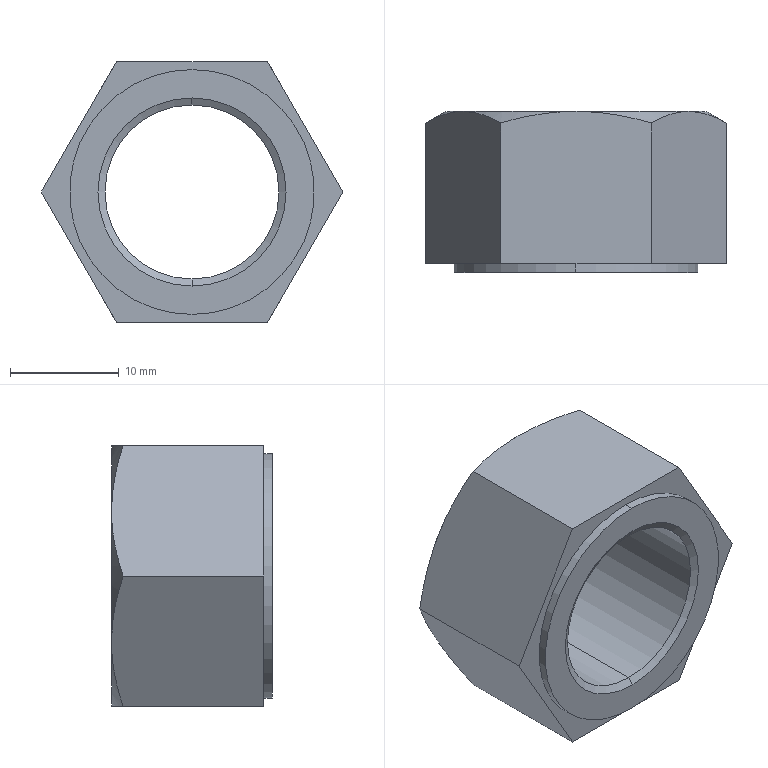Component | SolidWorks | GB_T6170-2015[Type1HexNutM16]-1 | 1 solid | 23 faces | box 27.71 x 14.8 x 24 mm | volume 4298 mm3 | cone 10 | plane 9 | cylinder 4 | commonest cylinder face diameters 22.5 x2 16 x2
STEP:
#1=COLOUR_RGB('',0.7922,0.8196,0.9333);
#2=FILL_AREA_STYLE_COLOUR('',#1);
#3=FILL_AREA_STYLE('',(#2));
#4=SURFACE_STYLE_FILL_AREA(#3);
#5=SURFACE_SIDE_STYLE('',(#4));
#6=SURFACE_STYLE_USAGE(.BOTH.,#5);
#7=PRESENTATION_STYLE_ASSIGNMENT((#6));
#8=CARTESIAN_POINT('',(5.257,-7.433,24.065));
#9=VERTEX_POINT('',#8);
#10=CARTESIAN_POINT('',(5.257,-7.433,23.179));
#11=VERTEX_POINT('',#10);
#12=CARTESIAN_POINT('',(5.257,-7.433,23.622));
#13=DIRECTION('',(-0.,1.,0.));
#14=DIRECTION('',(-0.,-0.,1.));
#15=AXIS2_PLACEMENT_3D('',#12,#13,#14);
#16=CIRCLE('',#15,0.4429);
#17=EDGE_CURVE('',#9,#11,#16,.T.);
#18=ORIENTED_EDGE('',*,*,#17,.T.);
#19=CARTESIAN_POINT('',(5.257,-7.401,23.179));
#20=VERTEX_POINT('',#19);
#21=CARTESIAN_POINT('',(5.257,-6.85,23.179));
#22=DIRECTION('',(-0.,1.,0.));
#23=VECTOR('',#22,39.37);
#24=LINE('',#21,#23);
#25=EDGE_CURVE('',#11,#20,#24,.T.);
#26=ORIENTED_EDGE('',*,*,#25,.T.);
#27=CARTESIAN_POINT('',(5.257,-7.401,24.065));
#28=VERTEX_POINT('',#27);
#29=CARTESIAN_POINT('',(5.257,-7.401,23.622));
#30=DIRECTION('',(-0.,1.,0.));
#31=DIRECTION('',(-0.,-0.,1.));
#32=AXIS2_PLACEMENT_3D('',#29,#30,#31);
#33=CIRCLE('',#32,0.4429);
#34=EDGE_CURVE('',#28,#20,#33,.T.);
#35=ORIENTED_EDGE('',*,*,#34,.F.);
#36=CARTESIAN_POINT('',(5.257,-6.85,24.065));
#37=DIRECTION('',(-0.,1.,0.));
#38=VECTOR('',#37,39.37);
#39=LINE('',#36,#38);
#40=EDGE_CURVE('',#9,#28,#39,.T.);
#41=ORIENTED_EDGE('',*,*,#40,.F.);
#42=EDGE_LOOP('',(#18,#26,#35,#41));
#43=FACE_OUTER_BOUND('',#42,.T.);
#44=CARTESIAN_POINT('',(5.257,-6.85,23.622));
#45=DIRECTION('',(-0.,1.,0.));
#46=DIRECTION('',(-0.,-0.,1.));
#47=AXIS2_PLACEMENT_3D('',#44,#45,#46);
#48=CYLINDRICAL_SURFACE('',#47,0.4429);
#49=ADVANCED_FACE('',(#43),#48,.T.);
#50=CARTESIAN_POINT('',(5.257,-7.418,23.307));
#51=VERTEX_POINT('',#50);
#52=CARTESIAN_POINT('',(5.257,-7.418,23.937));
#53=VERTEX_POINT('',#52);
#54=CARTESIAN_POINT('',(5.257,-7.418,23.622));
#55=DIRECTION('',(-0.,1.,0.));
#56=DIRECTION('',(0.,0.,-1.));
#57=AXIS2_PLACEMENT_3D('',#54,#55,#56);
#58=CIRCLE('',#57,0.315);
#59=EDGE_CURVE('',#51,#53,#58,.T.);
#60=ORIENTED_EDGE('',*,*,#59,.T.);
#61=CARTESIAN_POINT('',(5.257,-7.433,23.963));
#62=VERTEX_POINT('',#61);
#63=CARTESIAN_POINT('',(5.257,-7.433,23.963));
#64=DIRECTION('',(-0.,-0.5,0.866));
#65=VECTOR('',#64,39.37);
#66=LINE('',#63,#65);
#67=EDGE_CURVE('',#53,#62,#66,.T.);
#68=ORIENTED_EDGE('',*,*,#67,.T.);
#69=CARTESIAN_POINT('',(5.257,-7.433,23.281));
#70=VERTEX_POINT('',#69);
#71=CARTESIAN_POINT('',(5.257,-7.433,23.622));
#72=DIRECTION('',(-0.,1.,0.));
#73=DIRECTION('',(-0.,-0.,1.));
#74=AXIS2_PLACEMENT_3D('',#71,#72,#73);
#75=CIRCLE('',#74,0.3406);
#76=EDGE_CURVE('',#70,#62,#75,.T.);
#77=ORIENTED_EDGE('',*,*,#76,.F.);
#78=CARTESIAN_POINT('',(5.257,-7.433,23.281));
#79=DIRECTION('',(0.,-0.5,-0.866));
#80=VECTOR('',#79,39.37);
#81=LINE('',#78,#80);
#82=EDGE_CURVE('',#51,#70,#81,.T.);
#83=ORIENTED_EDGE('',*,*,#82,.F.);
#84=EDGE_LOOP('',(#60,#68,#77,#83));
#85=FACE_OUTER_BOUND('',#84,.T.);
#86=CARTESIAN_POINT('',(5.257,-7.433,23.622));
#87=DIRECTION('',(0.,-1.,-0.));
#88=DIRECTION('',(0.,0.,-1.));
#89=AXIS2_PLACEMENT_3D('',#86,#87,#88);
#90=CONICAL_SURFACE('',#89,0.3406,1.047);
#91=ADVANCED_FACE('',(#85),#90,.F.);
#92=CARTESIAN_POINT('',(5.257,-6.865,23.937));
#93=VERTEX_POINT('',#92);
#94=CARTESIAN_POINT('',(5.257,-6.865,23.307));
#95=VERTEX_POINT('',#94);
#96=CARTESIAN_POINT('',(5.257,-6.865,23.622));
#97=DIRECTION('',(0.,-1.,-0.));
#98=DIRECTION('',(-0.,-0.,1.));
#99=AXIS2_PLACEMENT_3D('',#96,#97,#98);
#100=CIRCLE('',#99,0.315);
#101=EDGE_CURVE('',#93,#95,#100,.T.);
#102=ORIENTED_EDGE('',*,*,#101,.T.);
#103=CARTESIAN_POINT('',(5.257,-6.85,23.281));
#104=VERTEX_POINT('',#103);
#105=CARTESIAN_POINT('',(5.257,-6.889,23.35));
#106=DIRECTION('',(0.,0.5,-0.866));
#107=VECTOR('',#106,39.37);
#108=LINE('',#105,#107);
#109=EDGE_CURVE('',#95,#104,#108,.T.);
#110=ORIENTED_EDGE('',*,*,#109,.T.);
#111=CARTESIAN_POINT('',(5.257,-6.85,23.963));
#112=VERTEX_POINT('',#111);
#113=CARTESIAN_POINT('',(5.257,-6.85,23.622));
#114=DIRECTION('',(-0.,1.,0.));
#115=DIRECTION('',(-0.,-0.,1.));
#116=AXIS2_PLACEMENT_3D('',#113,#114,#115);
#117=CIRCLE('',#116,0.3406);
#118=EDGE_CURVE('',#104,#112,#117,.T.);
#119=ORIENTED_EDGE('',*,*,#118,.T.);
#120=CARTESIAN_POINT('',(5.257,-6.889,23.894));
#121=DIRECTION('',(-0.,0.5,0.866));
#122=VECTOR('',#121,39.37);
#123=LINE('',#120,#122);
#124=EDGE_CURVE('',#93,#112,#123,.T.);
#125=ORIENTED_EDGE('',*,*,#124,.F.);
#126=EDGE_LOOP('',(#102,#110,#119,#125));
#127=FACE_OUTER_BOUND('',#126,.T.);
#128=CARTESIAN_POINT('',(5.257,-6.889,23.622));
#129=DIRECTION('',(-0.,1.,0.));
#130=DIRECTION('',(-0.,-0.,1.));
#131=AXIS2_PLACEMENT_3D('',#128,#129,#130);
#132=CONICAL_SURFACE('',#131,0.2723,1.047);
#133=ADVANCED_FACE('',(#127),#132,.F.);
#134=ORIENTED_EDGE('',*,*,#59,.F.);
#135=CARTESIAN_POINT('',(5.257,-7.433,23.307));
#136=DIRECTION('',(-0.,1.,0.));
#137=VECTOR('',#136,39.37);
#138=LINE('',#135,#137);
#139=EDGE_CURVE('',#51,#95,#138,.T.);
#140=ORIENTED_EDGE('',*,*,#139,.T.);
#141=ORIENTED_EDGE('',*,*,#101,.F.);
#142=CARTESIAN_POINT('',(5.257,-7.433,23.937));
#143=DIRECTION('',(-0.,1.,0.));
#144=VECTOR('',#143,39.37);
#145=LINE('',#142,#144);
#146=EDGE_CURVE('',#53,#93,#145,.T.);
#147=ORIENTED_EDGE('',*,*,#146,.F.);
#148=EDGE_LOOP('',(#134,#140,#141,#147));
#149=FACE_OUTER_BOUND('',#148,.T.);
#150=CARTESIAN_POINT('',(5.257,-7.433,23.622));
#151=DIRECTION('',(-0.,1.,0.));
#152=DIRECTION('',(-0.,-0.,1.));
#153=AXIS2_PLACEMENT_3D('',#150,#151,#152);
#154=CYLINDRICAL_SURFACE('',#153,0.315);
#155=ADVANCED_FACE('',(#149),#154,.F.);
#156=CARTESIAN_POINT('',(5.53,-7.401,24.094));
#157=VERTEX_POINT('',#156);
#158=CARTESIAN_POINT('',(5.53,-6.892,24.094));
#159=VERTEX_POINT('',#158);
#160=CARTESIAN_POINT('',(5.53,-7.433,24.094));
#161=DIRECTION('',(-0.,1.,0.));
#162=VECTOR('',#161,39.37);
#163=LINE('',#160,#162);
#164=EDGE_CURVE('',#157,#159,#163,.T.);
#165=ORIENTED_EDGE('',*,*,#164,.F.);
#166=CARTESIAN_POINT('',(5.803,-7.401,23.622));
#167=VERTEX_POINT('',#166);
#168=CARTESIAN_POINT('',(5.53,-7.401,24.094));
#169=DIRECTION('',(0.5,0.,-0.866));
#170=VECTOR('',#169,39.37);
#171=LINE('',#168,#170);
#172=EDGE_CURVE('',#157,#167,#171,.T.);
#173=ORIENTED_EDGE('',*,*,#172,.T.);
#174=CARTESIAN_POINT('',(5.803,-6.892,23.622));
#175=VERTEX_POINT('',#174);
#176=CARTESIAN_POINT('',(5.803,-7.433,23.622));
#177=DIRECTION('',(-0.,1.,0.));
#178=VECTOR('',#177,39.37);
#179=LINE('',#176,#178);
#180=EDGE_CURVE('',#167,#175,#179,.T.);
#181=ORIENTED_EDGE('',*,*,#180,.T.);
#182=CARTESIAN_POINT('',(5.666,-6.85,23.858));
#183=VERTEX_POINT('',#182);
#184=CARTESIAN_POINT('',(5.803,-6.892,23.622));
#185=CARTESIAN_POINT('',(5.78,-6.879,23.661));
#186=CARTESIAN_POINT('',(5.758,-6.869,23.7));
#187=CARTESIAN_POINT('',(5.712,-6.854,23.778));
#188=CARTESIAN_POINT('',(5.689,-6.85,23.818));
#189=CARTESIAN_POINT('',(5.666,-6.85,23.858));
#190=B_SPLINE_CURVE_WITH_KNOTS('',3,(#184,#185,#186,#187,#188,#189),.UNSPECIFIED.,.F.,.F.,(4,2,4),(0.00000024,0.003505,0.00701),.UNSPECIFIED.);
#191=EDGE_CURVE('',#175,#183,#190,.T.);
#192=ORIENTED_EDGE('',*,*,#191,.T.);
#193=CARTESIAN_POINT('',(5.666,-6.85,23.858));
#194=CARTESIAN_POINT('',(5.655,-6.85,23.878));
#195=CARTESIAN_POINT('',(5.643,-6.851,23.898));
#196=CARTESIAN_POINT('',(5.62,-6.855,23.938));
#197=CARTESIAN_POINT('',(5.609,-6.858,23.958));
#198=CARTESIAN_POINT('',(5.575,-6.869,24.017));
#199=CARTESIAN_POINT('',(5.552,-6.879,24.056));
#200=CARTESIAN_POINT('',(5.53,-6.892,24.094));
#201=B_SPLINE_CURVE_WITH_KNOTS('',3,(#193,#194,#195,#196,#197,#198,#199,#200),.UNSPECIFIED.,.F.,.F.,(4,2,2,4),(0.00701,0.008756,0.0105,0.01399),.UNSPECIFIED.);
#202=EDGE_CURVE('',#183,#159,#201,.T.);
#203=ORIENTED_EDGE('',*,*,#202,.T.);
#204=EDGE_LOOP('',(#165,#173,#181,#192,#203));
#205=FACE_OUTER_BOUND('',#204,.T.);
#206=CARTESIAN_POINT('',(5.53,-7.433,24.094));
#207=DIRECTION('',(0.866,0.,0.5));
#208=DIRECTION('',(0.5,0.,-0.866));
#209=AXIS2_PLACEMENT_3D('',#206,#207,#208);
#210=PLANE('',#209);
#211=ADVANCED_FACE('',(#205),#210,.T.);
#212=CARTESIAN_POINT('',(4.984,-7.401,24.094));
#213=VERTEX_POINT('',#212);
#214=CARTESIAN_POINT('',(4.984,-6.892,24.094));
#215=VERTEX_POINT('',#214);
#216=CARTESIAN_POINT('',(4.984,-7.433,24.094));
#217=DIRECTION('',(-0.,1.,0.));
#218=VECTOR('',#217,39.37);
#219=LINE('',#216,#218);
#220=EDGE_CURVE('',#213,#215,#219,.T.);
#221=ORIENTED_EDGE('',*,*,#220,.F.);
#222=CARTESIAN_POINT('',(4.984,-7.401,24.094));
#223=DIRECTION('',(1.,0.,0.));
#224=VECTOR('',#223,39.37);
#225=LINE('',#222,#224);
#226=EDGE_CURVE('',#213,#157,#225,.T.);
#227=ORIENTED_EDGE('',*,*,#226,.T.);
#228=ORIENTED_EDGE('',*,*,#164,.T.);
#229=CARTESIAN_POINT('',(5.257,-6.85,24.094));
#230=VERTEX_POINT('',#229);
#231=CARTESIAN_POINT('',(5.53,-6.892,24.094));
#232=CARTESIAN_POINT('',(5.486,-6.879,24.094));
#233=CARTESIAN_POINT('',(5.441,-6.869,24.094));
#234=CARTESIAN_POINT('',(5.373,-6.858,24.094));
#235=CARTESIAN_POINT('',(5.35,-6.855,24.094));
#236=CARTESIAN_POINT('',(5.303,-6.851,24.094));
#237=CARTESIAN_POINT('',(5.28,-6.85,24.094));
#238=CARTESIAN_POINT('',(5.257,-6.85,24.094));
#239=B_SPLINE_CURVE_WITH_KNOTS('',3,(#231,#232,#233,#234,#235,#236,#237,#238),.UNSPECIFIED.,.F.,.F.,(4,2,2,4),(0.03088,0.03439,0.03615,0.0379),.UNSPECIFIED.);
#240=EDGE_CURVE('',#159,#230,#239,.T.);
#241=ORIENTED_EDGE('',*,*,#240,.T.);
#242=CARTESIAN_POINT('',(5.257,-6.85,24.094));
#243=CARTESIAN_POINT('',(5.211,-6.85,24.094));
#244=CARTESIAN_POINT('',(5.165,-6.854,24.094));
#245=CARTESIAN_POINT('',(5.074,-6.869,24.094));
#246=CARTESIAN_POINT('',(5.029,-6.879,24.094));
#247=CARTESIAN_POINT('',(4.984,-6.892,24.094));
#248=B_SPLINE_CURVE_WITH_KNOTS('',3,(#242,#243,#244,#245,#246,#247),.UNSPECIFIED.,.F.,.F.,(4,2,4),(0.0379,0.04141,0.04492),.UNSPECIFIED.);
#249=EDGE_CURVE('',#230,#215,#248,.T.);
#250=ORIENTED_EDGE('',*,*,#249,.T.);
#251=EDGE_LOOP('',(#221,#227,#228,#241,#250));
#252=FACE_OUTER_BOUND('',#251,.T.);
#253=CARTESIAN_POINT('',(4.984,-7.433,24.094));
#254=DIRECTION('',(-0.,-0.,1.));
#255=DIRECTION('',(0.,-1.,-0.));
#256=AXIS2_PLACEMENT_3D('',#253,#254,#255);
#257=PLANE('',#256);
#258=ADVANCED_FACE('',(#252),#257,.T.);
#259=CARTESIAN_POINT('',(4.712,-7.401,23.622));
#260=VERTEX_POINT('',#259);
#261=CARTESIAN_POINT('',(4.712,-6.892,23.622));
#262=VERTEX_POINT('',#261);
#263=CARTESIAN_POINT('',(4.712,-7.433,23.622));
#264=DIRECTION('',(-0.,1.,0.));
#265=VECTOR('',#264,39.37);
#266=LINE('',#263,#265);
#267=EDGE_CURVE('',#260,#262,#266,.T.);
#268=ORIENTED_EDGE('',*,*,#267,.F.);
#269=CARTESIAN_POINT('',(4.712,-7.401,23.622));
#270=DIRECTION('',(0.5,0.,0.866));
#271=VECTOR('',#270,39.37);
#272=LINE('',#269,#271);
#273=EDGE_CURVE('',#260,#213,#272,.T.);
#274=ORIENTED_EDGE('',*,*,#273,.T.);
#275=ORIENTED_EDGE('',*,*,#220,.T.);
#276=CARTESIAN_POINT('',(4.848,-6.85,23.858));
#277=VERTEX_POINT('',#276);
#278=CARTESIAN_POINT('',(4.984,-6.892,24.094));
#279=CARTESIAN_POINT('',(4.962,-6.879,24.056));
#280=CARTESIAN_POINT('',(4.94,-6.869,24.017));
#281=CARTESIAN_POINT('',(4.894,-6.854,23.938));
#282=CARTESIAN_POINT('',(4.871,-6.85,23.899));
#283=CARTESIAN_POINT('',(4.848,-6.85,23.858));
#284=B_SPLINE_CURVE_WITH_KNOTS('',3,(#278,#279,#280,#281,#282,#283),.UNSPECIFIED.,.F.,.F.,(4,2,4),(0.00000024,0.003505,0.00701),.UNSPECIFIED.);
#285=EDGE_CURVE('',#215,#277,#284,.T.);
#286=ORIENTED_EDGE('',*,*,#285,.T.);
#287=CARTESIAN_POINT('',(4.848,-6.85,23.858));
#288=CARTESIAN_POINT('',(4.836,-6.85,23.838));
#289=CARTESIAN_POINT('',(4.825,-6.851,23.818));
#290=CARTESIAN_POINT('',(4.802,-6.855,23.778));
#291=CARTESIAN_POINT('',(4.79,-6.858,23.758));
#292=CARTESIAN_POINT('',(4.756,-6.869,23.699));
#293=CARTESIAN_POINT('',(4.734,-6.879,23.661));
#294=CARTESIAN_POINT('',(4.712,-6.892,23.622));
#295=B_SPLINE_CURVE_WITH_KNOTS('',3,(#287,#288,#289,#290,#291,#292,#293,#294),.UNSPECIFIED.,.F.,.F.,(4,2,2,4),(0.00701,0.008756,0.0105,0.01399),.UNSPECIFIED.);
#296=EDGE_CURVE('',#277,#262,#295,.T.);
#297=ORIENTED_EDGE('',*,*,#296,.T.);
#298=EDGE_LOOP('',(#268,#274,#275,#286,#297));
#299=FACE_OUTER_BOUND('',#298,.T.);
#300=CARTESIAN_POINT('',(4.712,-7.433,23.622));
#301=DIRECTION('',(-0.866,-0.,0.5));
#302=DIRECTION('',(0.5,0.,0.866));
#303=AXIS2_PLACEMENT_3D('',#300,#301,#302);
#304=PLANE('',#303);
#305=ADVANCED_FACE('',(#299),#304,.T.);
#306=CARTESIAN_POINT('',(4.984,-7.401,23.15));
#307=VERTEX_POINT('',#306);
#308=CARTESIAN_POINT('',(4.984,-6.892,23.15));
#309=VERTEX_POINT('',#308);
#310=CARTESIAN_POINT('',(4.984,-7.433,23.15));
#311=DIRECTION('',(-0.,1.,0.));
#312=VECTOR('',#311,39.37);
#313=LINE('',#310,#312);
#314=EDGE_CURVE('',#307,#309,#313,.T.);
#315=ORIENTED_EDGE('',*,*,#314,.F.);
#316=CARTESIAN_POINT('',(4.984,-7.401,23.15));
#317=DIRECTION('',(-0.5,-0.,0.866));
#318=VECTOR('',#317,39.37);
#319=LINE('',#316,#318);
#320=EDGE_CURVE('',#307,#260,#319,.T.);
#321=ORIENTED_EDGE('',*,*,#320,.T.);
#322=ORIENTED_EDGE('',*,*,#267,.T.);
#323=CARTESIAN_POINT('',(4.848,-6.85,23.386));
#324=VERTEX_POINT('',#323);
#325=CARTESIAN_POINT('',(4.712,-6.892,23.622));
#326=CARTESIAN_POINT('',(4.734,-6.879,23.583));
#327=CARTESIAN_POINT('',(4.756,-6.869,23.544));
#328=CARTESIAN_POINT('',(4.802,-6.854,23.466));
#329=CARTESIAN_POINT('',(4.825,-6.85,23.426));
#330=CARTESIAN_POINT('',(4.848,-6.85,23.386));
#331=B_SPLINE_CURVE_WITH_KNOTS('',3,(#325,#326,#327,#328,#329,#330),.UNSPECIFIED.,.F.,.F.,(4,2,4),(0.00000024,0.003505,0.00701),.UNSPECIFIED.);
#332=EDGE_CURVE('',#262,#324,#331,.T.);
#333=ORIENTED_EDGE('',*,*,#332,.T.);
#334=CARTESIAN_POINT('',(4.848,-6.85,23.386));
#335=CARTESIAN_POINT('',(4.859,-6.85,23.366));
#336=CARTESIAN_POINT('',(4.871,-6.851,23.346));
#337=CARTESIAN_POINT('',(4.894,-6.855,23.306));
#338=CARTESIAN_POINT('',(4.906,-6.858,23.286));
#339=CARTESIAN_POINT('',(4.94,-6.869,23.227));
#340=CARTESIAN_POINT('',(4.962,-6.879,23.188));
#341=CARTESIAN_POINT('',(4.984,-6.892,23.15));
#342=B_SPLINE_CURVE_WITH_KNOTS('',3,(#334,#335,#336,#337,#338,#339,#340,#341),.UNSPECIFIED.,.F.,.F.,(4,2,2,4),(0.00701,0.008756,0.0105,0.01399),.UNSPECIFIED.);
#343=EDGE_CURVE('',#324,#309,#342,.T.);
#344=ORIENTED_EDGE('',*,*,#343,.T.);
#345=EDGE_LOOP('',(#315,#321,#322,#333,#344));
#346=FACE_OUTER_BOUND('',#345,.T.);
#347=CARTESIAN_POINT('',(4.984,-7.433,23.15));
#348=DIRECTION('',(-0.866,-0.,-0.5));
#349=DIRECTION('',(-0.5,-0.,0.866));
#350=AXIS2_PLACEMENT_3D('',#347,#348,#349);
#351=PLANE('',#350);
#352=ADVANCED_FACE('',(#346),#351,.T.);
#353=CARTESIAN_POINT('',(5.53,-7.401,23.15));
#354=VERTEX_POINT('',#353);
#355=CARTESIAN_POINT('',(5.53,-6.892,23.15));
#356=VERTEX_POINT('',#355);
#357=CARTESIAN_POINT('',(5.53,-7.433,23.15));
#358=DIRECTION('',(-0.,1.,0.));
#359=VECTOR('',#358,39.37);
#360=LINE('',#357,#359);
#361=EDGE_CURVE('',#354,#356,#360,.T.);
#362=ORIENTED_EDGE('',*,*,#361,.F.);
#363=CARTESIAN_POINT('',(5.53,-7.401,23.15));
#364=DIRECTION('',(-1.,-0.,-0.));
#365=VECTOR('',#364,39.37);
#366=LINE('',#363,#365);
#367=EDGE_CURVE('',#354,#307,#366,.T.);
#368=ORIENTED_EDGE('',*,*,#367,.T.);
#369=ORIENTED_EDGE('',*,*,#314,.T.);
#370=CARTESIAN_POINT('',(5.257,-6.85,23.15));
#371=VERTEX_POINT('',#370);
#372=CARTESIAN_POINT('',(4.984,-6.892,23.15));
#373=CARTESIAN_POINT('',(5.029,-6.879,23.15));
#374=CARTESIAN_POINT('',(5.074,-6.869,23.15));
#375=CARTESIAN_POINT('',(5.165,-6.854,23.15));
#376=CARTESIAN_POINT('',(5.211,-6.85,23.15));
#377=CARTESIAN_POINT('',(5.257,-6.85,23.15));
#378=B_SPLINE_CURVE_WITH_KNOTS('',3,(#372,#373,#374,#375,#376,#377),.UNSPECIFIED.,.F.,.F.,(4,2,4),(0.01255,0.01606,0.01957),.UNSPECIFIED.);
#379=EDGE_CURVE('',#309,#371,#378,.T.);
#380=ORIENTED_EDGE('',*,*,#379,.T.);
#381=CARTESIAN_POINT('',(5.257,-6.85,23.15));
#382=CARTESIAN_POINT('',(5.28,-6.85,23.15));
#383=CARTESIAN_POINT('',(5.303,-6.851,23.15));
#384=CARTESIAN_POINT('',(5.35,-6.855,23.15));
#385=CARTESIAN_POINT('',(5.373,-6.858,23.15));
#386=CARTESIAN_POINT('',(5.441,-6.869,23.15));
#387=CARTESIAN_POINT('',(5.486,-6.879,23.15));
#388=CARTESIAN_POINT('',(5.53,-6.892,23.15));
#389=B_SPLINE_CURVE_WITH_KNOTS('',3,(#381,#382,#383,#384,#385,#386,#387,#388),.UNSPECIFIED.,.F.,.F.,(4,2,2,4),(0.01957,0.02132,0.02307,0.02658),.UNSPECIFIED.);
#390=EDGE_CURVE('',#371,#356,#389,.T.);
#391=ORIENTED_EDGE('',*,*,#390,.T.);
#392=EDGE_LOOP('',(#362,#368,#369,#380,#391));
#393=FACE_OUTER_BOUND('',#392,.T.);
#394=CARTESIAN_POINT('',(5.53,-7.433,23.15));
#395=DIRECTION('',(0.,0.,-1.));
#396=DIRECTION('',(-0.,1.,0.));
#397=AXIS2_PLACEMENT_3D('',#394,#395,#396);
#398=PLANE('',#397);
#399=ADVANCED_FACE('',(#393),#398,.T.);
#400=ORIENTED_EDGE('',*,*,#180,.F.);
#401=CARTESIAN_POINT('',(5.803,-7.401,23.622));
#402=DIRECTION('',(-0.5,-0.,-0.866));
#403=VECTOR('',#402,39.37);
#404=LINE('',#401,#403);
#405=EDGE_CURVE('',#167,#354,#404,.T.);
#406=ORIENTED_EDGE('',*,*,#405,.T.);
#407=ORIENTED_EDGE('',*,*,#361,.T.);
#408=CARTESIAN_POINT('',(5.666,-6.85,23.386));
#409=VERTEX_POINT('',#408);
#410=CARTESIAN_POINT('',(5.53,-6.892,23.15));
#411=CARTESIAN_POINT('',(5.552,-6.879,23.188));
#412=CARTESIAN_POINT('',(5.575,-6.869,23.227));
#413=CARTESIAN_POINT('',(5.62,-6.854,23.306));
#414=CARTESIAN_POINT('',(5.643,-6.85,23.346));
#415=CARTESIAN_POINT('',(5.666,-6.85,23.386));
#416=B_SPLINE_CURVE_WITH_KNOTS('',3,(#410,#411,#412,#413,#414,#415),.UNSPECIFIED.,.F.,.F.,(4,2,4),(0.00000024,0.003505,0.00701),.UNSPECIFIED.);
#417=EDGE_CURVE('',#356,#409,#416,.T.);
#418=ORIENTED_EDGE('',*,*,#417,.T.);
#419=CARTESIAN_POINT('',(5.666,-6.85,23.386));
#420=CARTESIAN_POINT('',(5.678,-6.85,23.406));
#421=CARTESIAN_POINT('',(5.689,-6.851,23.426));
#422=CARTESIAN_POINT('',(5.712,-6.855,23.466));
#423=CARTESIAN_POINT('',(5.724,-6.858,23.486));
#424=CARTESIAN_POINT('',(5.758,-6.869,23.545));
#425=CARTESIAN_POINT('',(5.78,-6.879,23.584));
#426=CARTESIAN_POINT('',(5.803,-6.892,23.622));
#427=B_SPLINE_CURVE_WITH_KNOTS('',3,(#419,#420,#421,#422,#423,#424,#425,#426),.UNSPECIFIED.,.F.,.F.,(4,2,2,4),(0.00701,0.008756,0.0105,0.01399),.UNSPECIFIED.);
#428=EDGE_CURVE('',#409,#175,#427,.T.);
#429=ORIENTED_EDGE('',*,*,#428,.T.);
#430=EDGE_LOOP('',(#400,#406,#407,#418,#429));
#431=FACE_OUTER_BOUND('',#430,.T.);
#432=CARTESIAN_POINT('',(5.803,-7.433,23.622));
#433=DIRECTION('',(0.866,0.,-0.5));
#434=DIRECTION('',(-0.5,-0.,-0.866));
#435=AXIS2_PLACEMENT_3D('',#432,#433,#434);
#436=PLANE('',#435);
#437=ADVANCED_FACE('',(#431),#436,.T.);
#438=ORIENTED_EDGE('',*,*,#76,.T.);
#439=CARTESIAN_POINT('',(5.257,-7.433,23.622));
#440=DIRECTION('',(-0.,1.,0.));
#441=DIRECTION('',(-0.,-0.,1.));
#442=AXIS2_PLACEMENT_3D('',#439,#440,#441);
#443=CIRCLE('',#442,0.3406);
#444=EDGE_CURVE('',#62,#70,#443,.T.);
#445=ORIENTED_EDGE('',*,*,#444,.T.);
#446=EDGE_LOOP('',(#438,#445));
#447=FACE_BOUND('',#446,.T.);
#448=ORIENTED_EDGE('',*,*,#17,.F.);
#449=CARTESIAN_POINT('',(5.257,-7.433,23.622));
#450=DIRECTION('',(-0.,1.,0.));
#451=DIRECTION('',(-0.,-0.,1.));
#452=AXIS2_PLACEMENT_3D('',#449,#450,#451);
#453=CIRCLE('',#452,0.4429);
#454=EDGE_CURVE('',#11,#9,#453,.T.);
#455=ORIENTED_EDGE('',*,*,#454,.F.);
#456=EDGE_LOOP('',(#448,#455));
#457=FACE_OUTER_BOUND('',#456,.T.);
#458=CARTESIAN_POINT('',(5.803,-7.433,23.622));
#459=DIRECTION('',(-0.,1.,0.));
#460=DIRECTION('',(-0.,-0.,1.));
#461=AXIS2_PLACEMENT_3D('',#458,#459,#460);
#462=PLANE('',#461);
#463=ADVANCED_FACE('',(#447,#457),#462,.F.);
#464=CARTESIAN_POINT('',(5.257,-6.85,23.622));
#465=DIRECTION('',(-0.,1.,0.));
#466=DIRECTION('',(-0.,-0.,1.));
#467=AXIS2_PLACEMENT_3D('',#464,#465,#466);
#468=CIRCLE('',#467,0.3406);
#469=EDGE_CURVE('',#112,#104,#468,.T.);
#470=ORIENTED_EDGE('',*,*,#469,.F.);
#471=ORIENTED_EDGE('',*,*,#118,.F.);
#472=EDGE_LOOP('',(#470,#471));
#473=FACE_BOUND('',#472,.T.);
#474=CARTESIAN_POINT('',(5.257,-6.85,23.622));
#475=DIRECTION('',(-0.,1.,0.));
#476=DIRECTION('',(-0.,-0.,1.));
#477=AXIS2_PLACEMENT_3D('',#474,#475,#476);
#478=CIRCLE('',#477,0.4724);
#479=EDGE_CURVE('',#277,#230,#478,.T.);
#480=ORIENTED_EDGE('',*,*,#479,.T.);
#481=CARTESIAN_POINT('',(5.257,-6.85,23.622));
#482=DIRECTION('',(-0.,1.,0.));
#483=DIRECTION('',(-0.,-0.,1.));
#484=AXIS2_PLACEMENT_3D('',#481,#482,#483);
#485=CIRCLE('',#484,0.4724);
#486=EDGE_CURVE('',#230,#183,#485,.T.);
#487=ORIENTED_EDGE('',*,*,#486,.T.);
#488=CARTESIAN_POINT('',(5.257,-6.85,23.622));
#489=DIRECTION('',(-0.,1.,0.));
#490=DIRECTION('',(-0.,-0.,1.));
#491=AXIS2_PLACEMENT_3D('',#488,#489,#490);
#492=CIRCLE('',#491,0.4724);
#493=EDGE_CURVE('',#183,#409,#492,.T.);
#494=ORIENTED_EDGE('',*,*,#493,.T.);
#495=CARTESIAN_POINT('',(5.257,-6.85,23.622));
#496=DIRECTION('',(-0.,1.,0.));
#497=DIRECTION('',(-0.,-0.,1.));
#498=AXIS2_PLACEMENT_3D('',#495,#496,#497);
#499=CIRCLE('',#498,0.4724);
#500=EDGE_CURVE('',#409,#371,#499,.T.);
#501=ORIENTED_EDGE('',*,*,#500,.T.);
#502=CARTESIAN_POINT('',(5.257,-6.85,23.622));
#503=DIRECTION('',(-0.,1.,0.));
#504=DIRECTION('',(-0.,-0.,1.));
#505=AXIS2_PLACEMENT_3D('',#502,#503,#504);
#506=CIRCLE('',#505,0.4724);
#507=EDGE_CURVE('',#371,#324,#506,.T.);
#508=ORIENTED_EDGE('',*,*,#507,.T.);
#509=CARTESIAN_POINT('',(5.257,-6.85,23.622));
#510=DIRECTION('',(-0.,1.,0.));
#511=DIRECTION('',(-0.,-0.,1.));
#512=AXIS2_PLACEMENT_3D('',#509,#510,#511);
#513=CIRCLE('',#512,0.4724);
#514=EDGE_CURVE('',#324,#277,#513,.T.);
#515=ORIENTED_EDGE('',*,*,#514,.T.);
#516=EDGE_LOOP('',(#480,#487,#494,#501,#508,#515));
#517=FACE_OUTER_BOUND('',#516,.T.);
#518=CARTESIAN_POINT('',(5.803,-6.85,23.622));
#519=DIRECTION('',(-0.,1.,0.));
#520=DIRECTION('',(-0.,-0.,1.));
#521=AXIS2_PLACEMENT_3D('',#518,#519,#520);
#522=PLANE('',#521);
#523=ADVANCED_FACE('',(#473,#517),#522,.T.);
#524=ORIENTED_EDGE('',*,*,#139,.F.);
#525=CARTESIAN_POINT('',(5.257,-7.418,23.622));
#526=DIRECTION('',(-0.,1.,0.));
#527=DIRECTION('',(0.,0.,-1.));
#528=AXIS2_PLACEMENT_3D('',#525,#526,#527);
#529=CIRCLE('',#528,0.315);
#530=EDGE_CURVE('',#53,#51,#529,.T.);
#531=ORIENTED_EDGE('',*,*,#530,.F.);
#532=ORIENTED_EDGE('',*,*,#146,.T.);
#533=CARTESIAN_POINT('',(5.257,-6.865,23.622));
#534=DIRECTION('',(0.,-1.,-0.));
#535=DIRECTION('',(-0.,-0.,1.));
#536=AXIS2_PLACEMENT_3D('',#533,#534,#535);
#537=CIRCLE('',#536,0.315);
#538=EDGE_CURVE('',#95,#93,#537,.T.);
#539=ORIENTED_EDGE('',*,*,#538,.F.);
#540=EDGE_LOOP('',(#524,#531,#532,#539));
#541=FACE_OUTER_BOUND('',#540,.T.);
#542=CARTESIAN_POINT('',(5.257,-7.433,23.622));
#543=DIRECTION('',(-0.,1.,0.));
#544=DIRECTION('',(-0.,-0.,1.));
#545=AXIS2_PLACEMENT_3D('',#542,#543,#544);
#546=CYLINDRICAL_SURFACE('',#545,0.315);
#547=ADVANCED_FACE('',(#541),#546,.F.);
#548=ORIENTED_EDGE('',*,*,#109,.F.);
#549=ORIENTED_EDGE('',*,*,#538,.T.);
#550=ORIENTED_EDGE('',*,*,#124,.T.);
#551=ORIENTED_EDGE('',*,*,#469,.T.);
#552=EDGE_LOOP('',(#548,#549,#550,#551));
#553=FACE_OUTER_BOUND('',#552,.T.);
#554=CARTESIAN_POINT('',(5.257,-6.889,23.622));
#555=DIRECTION('',(-0.,1.,0.));
#556=DIRECTION('',(-0.,-0.,1.));
#557=AXIS2_PLACEMENT_3D('',#554,#555,#556);
#558=CONICAL_SURFACE('',#557,0.2723,1.047);
#559=ADVANCED_FACE('',(#553),#558,.F.);
#560=ORIENTED_EDGE('',*,*,#67,.F.);
#561=ORIENTED_EDGE('',*,*,#530,.T.);
#562=ORIENTED_EDGE('',*,*,#82,.T.);
#563=ORIENTED_EDGE('',*,*,#444,.F.);
#564=EDGE_LOOP('',(#560,#561,#562,#563));
#565=FACE_OUTER_BOUND('',#564,.T.);
#566=CARTESIAN_POINT('',(5.257,-7.433,23.622));
#567=DIRECTION('',(0.,-1.,-0.));
#568=DIRECTION('',(0.,0.,-1.));
#569=AXIS2_PLACEMENT_3D('',#566,#567,#568);
#570=CONICAL_SURFACE('',#569,0.3406,1.047);
#571=ADVANCED_FACE('',(#565),#570,.F.);
#572=ORIENTED_EDGE('',*,*,#428,.F.);
#573=ORIENTED_EDGE('',*,*,#493,.F.);
#574=ORIENTED_EDGE('',*,*,#191,.F.);
#575=EDGE_LOOP('',(#572,#573,#574));
#576=FACE_OUTER_BOUND('',#575,.T.);
#577=CARTESIAN_POINT('',(5.257,-6.85,23.622));
#578=DIRECTION('',(0.,-1.,-0.));
#579=DIRECTION('',(-0.,-0.,1.));
#580=AXIS2_PLACEMENT_3D('',#577,#578,#579);
#581=CONICAL_SURFACE('',#580,0.4724,1.047);
#582=ADVANCED_FACE('',(#576),#581,.T.);
#583=ORIENTED_EDGE('',*,*,#500,.F.);
#584=ORIENTED_EDGE('',*,*,#417,.F.);
#585=ORIENTED_EDGE('',*,*,#390,.F.);
#586=EDGE_LOOP('',(#583,#584,#585));
#587=FACE_OUTER_BOUND('',#586,.T.);
#588=CARTESIAN_POINT('',(5.257,-6.85,23.622));
#589=DIRECTION('',(0.,-1.,-0.));
#590=DIRECTION('',(-0.,-0.,1.));
#591=AXIS2_PLACEMENT_3D('',#588,#589,#590);
#592=CONICAL_SURFACE('',#591,0.4724,1.047);
#593=ADVANCED_FACE('',(#587),#592,.T.);
#594=ORIENTED_EDGE('',*,*,#507,.F.);
#595=ORIENTED_EDGE('',*,*,#379,.F.);
#596=ORIENTED_EDGE('',*,*,#343,.F.);
#597=EDGE_LOOP('',(#594,#595,#596));
#598=FACE_OUTER_BOUND('',#597,.T.);
#599=CARTESIAN_POINT('',(5.257,-6.85,23.622));
#600=DIRECTION('',(0.,-1.,-0.));
#601=DIRECTION('',(-0.,-0.,1.));
#602=AXIS2_PLACEMENT_3D('',#599,#600,#601);
#603=CONICAL_SURFACE('',#602,0.4724,1.047);
#604=ADVANCED_FACE('',(#598),#603,.T.);
#605=ORIENTED_EDGE('',*,*,#514,.F.);
#606=ORIENTED_EDGE('',*,*,#332,.F.);
#607=ORIENTED_EDGE('',*,*,#296,.F.);
#608=EDGE_LOOP('',(#605,#606,#607));
#609=FACE_OUTER_BOUND('',#608,.T.);
#610=CARTESIAN_POINT('',(5.257,-6.85,23.622));
#611=DIRECTION('',(0.,-1.,-0.));
#612=DIRECTION('',(-0.,-0.,1.));
#613=AXIS2_PLACEMENT_3D('',#610,#611,#612);
#614=CONICAL_SURFACE('',#613,0.4724,1.047);
#615=ADVANCED_FACE('',(#609),#614,.T.);
#616=ORIENTED_EDGE('',*,*,#479,.F.);
#617=ORIENTED_EDGE('',*,*,#285,.F.);
#618=ORIENTED_EDGE('',*,*,#249,.F.);
#619=EDGE_LOOP('',(#616,#617,#618));
#620=FACE_OUTER_BOUND('',#619,.T.);
#621=CARTESIAN_POINT('',(5.257,-6.85,23.622));
#622=DIRECTION('',(0.,-1.,-0.));
#623=DIRECTION('',(-0.,-0.,1.));
#624=AXIS2_PLACEMENT_3D('',#621,#622,#623);
#625=CONICAL_SURFACE('',#624,0.4724,1.047);
#626=ADVANCED_FACE('',(#620),#625,.T.);
#627=ORIENTED_EDGE('',*,*,#486,.F.);
#628=ORIENTED_EDGE('',*,*,#240,.F.);
#629=ORIENTED_EDGE('',*,*,#202,.F.);
#630=EDGE_LOOP('',(#627,#628,#629));
#631=FACE_OUTER_BOUND('',#630,.T.);
#632=CARTESIAN_POINT('',(5.257,-6.85,23.622));
#633=DIRECTION('',(0.,-1.,-0.));
#634=DIRECTION('',(-0.,-0.,1.));
#635=AXIS2_PLACEMENT_3D('',#632,#633,#634);
#636=CONICAL_SURFACE('',#635,0.4724,1.047);
#637=ADVANCED_FACE('',(#631),#636,.T.);
#638=ORIENTED_EDGE('',*,*,#25,.F.);
#639=ORIENTED_EDGE('',*,*,#454,.T.);
#640=ORIENTED_EDGE('',*,*,#40,.T.);
#641=CARTESIAN_POINT('',(5.257,-7.401,23.622));
#642=DIRECTION('',(-0.,1.,0.));
#643=DIRECTION('',(-0.,-0.,1.));
#644=AXIS2_PLACEMENT_3D('',#641,#642,#643);
#645=CIRCLE('',#644,0.4429);
#646=EDGE_CURVE('',#20,#28,#645,.T.);
#647=ORIENTED_EDGE('',*,*,#646,.F.);
#648=EDGE_LOOP('',(#638,#639,#640,#647));
#649=FACE_OUTER_BOUND('',#648,.T.);
#650=CARTESIAN_POINT('',(5.257,-6.85,23.622));
#651=DIRECTION('',(-0.,1.,0.));
#652=DIRECTION('',(-0.,-0.,1.));
#653=AXIS2_PLACEMENT_3D('',#650,#651,#652);
#654=CYLINDRICAL_SURFACE('',#653,0.4429);
#655=ADVANCED_FACE('',(#649),#654,.T.);
#656=ORIENTED_EDGE('',*,*,#34,.T.);
#657=ORIENTED_EDGE('',*,*,#646,.T.);
#658=EDGE_LOOP('',(#656,#657));
#659=FACE_BOUND('',#658,.T.);
#660=ORIENTED_EDGE('',*,*,#226,.F.);
#661=ORIENTED_EDGE('',*,*,#273,.F.);
#662=ORIENTED_EDGE('',*,*,#320,.F.);
#663=ORIENTED_EDGE('',*,*,#367,.F.);
#664=ORIENTED_EDGE('',*,*,#405,.F.);
#665=ORIENTED_EDGE('',*,*,#172,.F.);
#666=EDGE_LOOP('',(#660,#661,#662,#663,#664,#665));
#667=FACE_OUTER_BOUND('',#666,.T.);
#668=CARTESIAN_POINT('',(4.814,-7.401,23.622));
#669=DIRECTION('',(0.,-1.,-0.));
#670=DIRECTION('',(0.,0.,-1.));
#671=AXIS2_PLACEMENT_3D('',#668,#669,#670);
#672=PLANE('',#671);
#673=ADVANCED_FACE('',(#659,#667),#672,.T.);
#674=CLOSED_SHELL('',(#49,#91,#133,#155,#211,#258,#305,#352,#399,#437,#463,#523,#547,#559,#571,#582,#593,#604,#615,#626,#637,#655,#673));
#675=MANIFOLD_SOLID_BREP('',#674);
#676=STYLED_ITEM('',(#7),#675);
#677=PRESENTATION_LAYER_ASSIGNMENT('','',(#676));
#678=(LENGTH_UNIT()NAMED_UNIT(*)SI_UNIT($,.METRE.));
#679=LENGTH_MEASURE_WITH_UNIT(LENGTH_MEASURE(0.0254),#678);
#680=DIMENSIONAL_EXPONENTS(1.,0.,0.,0.,0.,0.,0.);
#681=(CONVERSION_BASED_UNIT('',#679)LENGTH_UNIT()NAMED_UNIT(#680));
#682=UNCERTAINTY_MEASURE_WITH_UNIT(LENGTH_MEASURE(0.00001),#681,'','');
#683=(NAMED_UNIT(*)PLANE_ANGLE_UNIT()SI_UNIT($,.RADIAN.));
#684=(NAMED_UNIT(*)SI_UNIT($,.STERADIAN.)SOLID_ANGLE_UNIT());
#685=(GEOMETRIC_REPRESENTATION_CONTEXT(3)GLOBAL_UNCERTAINTY_ASSIGNED_CONTEXT((#682))GLOBAL_UNIT_ASSIGNED_CONTEXT((#681,#683,#684))REPRESENTATION_CONTEXT('',''));
#686=MECHANICAL_DESIGN_GEOMETRIC_PRESENTATION_REPRESENTATION('',(#676),#685);
#687=CARTESIAN_POINT('',(0.,0.,0.));
#688=DIRECTION('',(0.,0.,1.));
#689=DIRECTION('',(1.,0.,0.));
#690=AXIS2_PLACEMENT_3D('',#687,#688,#689);
#691=(LENGTH_UNIT()NAMED_UNIT(*)SI_UNIT($,.METRE.));
#692=LENGTH_MEASURE_WITH_UNIT(LENGTH_MEASURE(0.0254),#691);
#693=DIMENSIONAL_EXPONENTS(1.,0.,0.,0.,0.,0.,0.);
#694=(CONVERSION_BASED_UNIT('',#692)LENGTH_UNIT()NAMED_UNIT(#693));
#695=UNCERTAINTY_MEASURE_WITH_UNIT(LENGTH_MEASURE(0.00001),#694,'','');
#696=(NAMED_UNIT(*)PLANE_ANGLE_UNIT()SI_UNIT($,.RADIAN.));
#697=(NAMED_UNIT(*)SI_UNIT($,.STERADIAN.)SOLID_ANGLE_UNIT());
#698=(GEOMETRIC_REPRESENTATION_CONTEXT(3)GLOBAL_UNCERTAINTY_ASSIGNED_CONTEXT((#695))GLOBAL_UNIT_ASSIGNED_CONTEXT((#694,#696,#697))REPRESENTATION_CONTEXT('',''));
#699=ADVANCED_BREP_SHAPE_REPRESENTATION('',(#675,#690),#698);